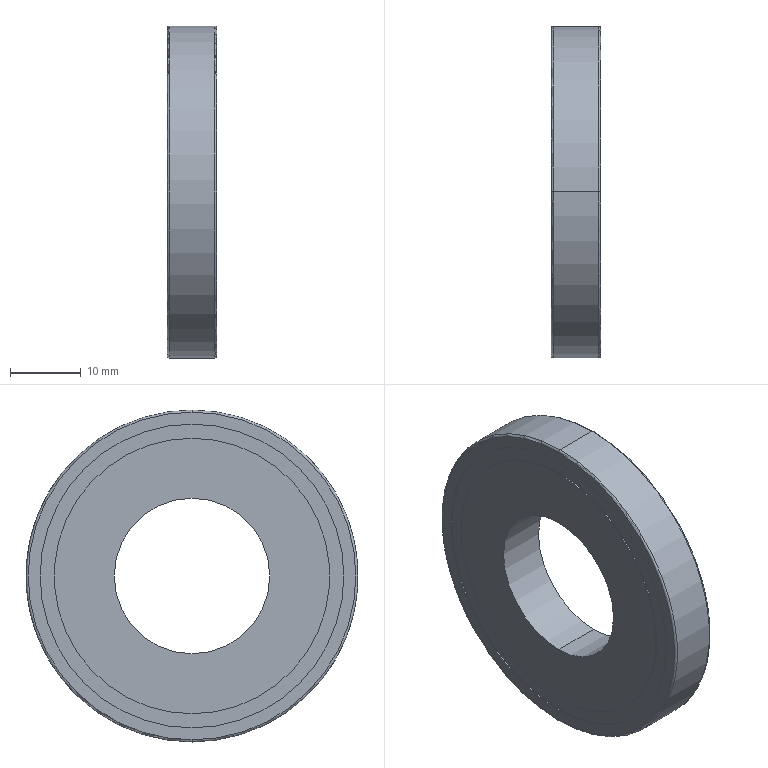Component | SolidWorks | DeepGrooveBallBearing16002-4 | 36 solids | 176 faces | volume 8155 mm3 | sphere 140 | cylinder 16 | torus 10 | plane 6 | cone 4 | commonest cylinder face diameters 39 x6 43 x6 22.02 x2 47 x2